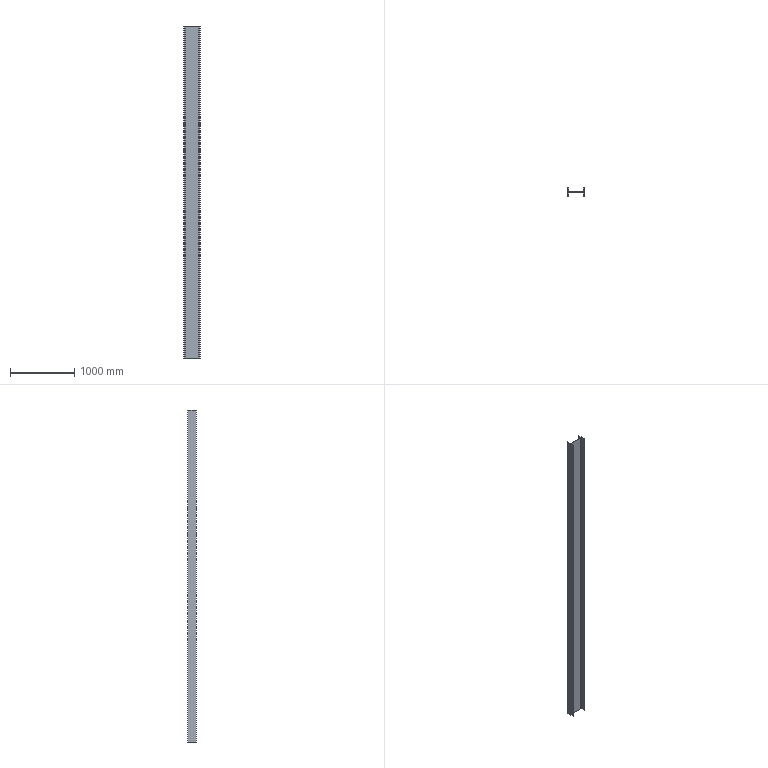Component | SolidWorks | H250X125-3800-1 | 1 solid | 18 faces | box 250 x 125 x 5180 mm | volume 19617027 mm3 | plane 14 | cylinder 4 | commonest cylinder face diameters 26 x4
build123d program:
from build123d import *

# Parameters (mm, degrees)
H_BEAM_HN250_125_1_DEPTH = 5180


with BuildPart() as part:
    # Sketch1 → H-Beam HN250_125_1 (new body)
    with BuildSketch(Plane.YZ):
        with BuildLine():
            Line((-62.5, -125), (-62.5, -116))
            Line((-62.5, -116), (-16, -116))
            ThreePointArc((-16, -116), (-6.808, -112.192), (-3, -103))
            Line((-3, -103), (-3, 103))
            ThreePointArc((-3, 103), (-6.808, 112.192), (-16, 116))
            Line((-16, 116), (-62.5, 116))
            Line((-62.5, 116), (-62.5, 125))
            Line((-62.5, 125), (62.5, 125))
            Line((62.5, 125), (62.5, 116))
            Line((62.5, 116), (16, 116))
            ThreePointArc((16, 116), (6.808, 112.192), (3, 103))
            Line((3, 103), (3, -103))
            ThreePointArc((3, -103), (6.808, -112.192), (16, -116))
            Line((16, -116), (62.5, -116))
            Line((62.5, -116), (62.5, -125))
            Line((62.5, -125), (-62.5, -125))
        make_face()
    extrude(amount=H_BEAM_HN250_125_1_DEPTH)


solid = part.part

# Placed as in the assembly
solid = solid.moved(Location((1944.926, 867.654, 5279), (0, 90, 0)))
STEP:
#1=COLOUR_RGB('',0.7922,0.8196,0.9333);
#2=FILL_AREA_STYLE_COLOUR('',#1);
#3=FILL_AREA_STYLE('',(#2));
#4=SURFACE_STYLE_FILL_AREA(#3);
#5=SURFACE_SIDE_STYLE('',(#4));
#6=SURFACE_STYLE_USAGE(.BOTH.,#5);
#7=PRESENTATION_STYLE_ASSIGNMENT((#6));
#8=CARTESIAN_POINT('',(71.651,31.699,207.835));
#9=VERTEX_POINT('',#8);
#10=CARTESIAN_POINT('',(71.651,36.62,207.835));
#11=VERTEX_POINT('',#10);
#12=CARTESIAN_POINT('',(71.651,36.62,207.835));
#13=DIRECTION('',(0.,1.,0.));
#14=VECTOR('',#13,39.37);
#15=LINE('',#12,#14);
#16=EDGE_CURVE('',#9,#11,#15,.T.);
#17=ORIENTED_EDGE('',*,*,#16,.T.);
#18=CARTESIAN_POINT('',(71.651,36.62,3.898));
#19=VERTEX_POINT('',#18);
#20=CARTESIAN_POINT('',(71.651,36.62,3.898));
#21=DIRECTION('',(0.,0.,1.));
#22=VECTOR('',#21,39.37);
#23=LINE('',#20,#22);
#24=EDGE_CURVE('',#19,#11,#23,.T.);
#25=ORIENTED_EDGE('',*,*,#24,.F.);
#26=CARTESIAN_POINT('',(71.651,31.699,3.898));
#27=VERTEX_POINT('',#26);
#28=CARTESIAN_POINT('',(71.651,36.62,3.898));
#29=DIRECTION('',(0.,1.,0.));
#30=VECTOR('',#29,39.37);
#31=LINE('',#28,#30);
#32=EDGE_CURVE('',#27,#19,#31,.T.);
#33=ORIENTED_EDGE('',*,*,#32,.F.);
#34=CARTESIAN_POINT('',(71.651,31.699,3.898));
#35=DIRECTION('',(0.,0.,1.));
#36=VECTOR('',#35,39.37);
#37=LINE('',#34,#36);
#38=EDGE_CURVE('',#27,#9,#37,.T.);
#39=ORIENTED_EDGE('',*,*,#38,.T.);
#40=EDGE_LOOP('',(#17,#25,#33,#39));
#41=FACE_OUTER_BOUND('',#40,.T.);
#42=CARTESIAN_POINT('',(71.651,36.62,3.898));
#43=DIRECTION('',(1.,0.,0.));
#44=DIRECTION('',(0.,0.,-1.));
#45=AXIS2_PLACEMENT_3D('',#42,#43,#44);
#46=PLANE('',#45);
#47=ADVANCED_FACE('',(#41),#46,.F.);
#48=CARTESIAN_POINT('',(72.005,36.62,207.835));
#49=VERTEX_POINT('',#48);
#50=CARTESIAN_POINT('',(72.005,36.62,207.835));
#51=DIRECTION('',(1.,0.,0.));
#52=VECTOR('',#51,39.37);
#53=LINE('',#50,#52);
#54=EDGE_CURVE('',#11,#49,#53,.T.);
#55=ORIENTED_EDGE('',*,*,#54,.T.);
#56=CARTESIAN_POINT('',(72.005,36.62,3.898));
#57=VERTEX_POINT('',#56);
#58=CARTESIAN_POINT('',(72.005,36.62,3.898));
#59=DIRECTION('',(0.,0.,1.));
#60=VECTOR('',#59,39.37);
#61=LINE('',#58,#60);
#62=EDGE_CURVE('',#57,#49,#61,.T.);
#63=ORIENTED_EDGE('',*,*,#62,.F.);
#64=CARTESIAN_POINT('',(72.005,36.62,3.898));
#65=DIRECTION('',(1.,0.,0.));
#66=VECTOR('',#65,39.37);
#67=LINE('',#64,#66);
#68=EDGE_CURVE('',#19,#57,#67,.T.);
#69=ORIENTED_EDGE('',*,*,#68,.F.);
#70=ORIENTED_EDGE('',*,*,#24,.T.);
#71=EDGE_LOOP('',(#55,#63,#69,#70));
#72=FACE_OUTER_BOUND('',#71,.T.);
#73=CARTESIAN_POINT('',(72.005,36.62,3.898));
#74=DIRECTION('',(0.,-1.,0.));
#75=DIRECTION('',(-1.,0.,0.));
#76=AXIS2_PLACEMENT_3D('',#73,#74,#75);
#77=PLANE('',#76);
#78=ADVANCED_FACE('',(#72),#77,.F.);
#79=CARTESIAN_POINT('',(72.005,34.79,207.835));
#80=VERTEX_POINT('',#79);
#81=CARTESIAN_POINT('',(72.005,36.62,207.835));
#82=DIRECTION('',(0.,-1.,0.));
#83=VECTOR('',#82,39.37);
#84=LINE('',#81,#83);
#85=EDGE_CURVE('',#49,#80,#84,.T.);
#86=ORIENTED_EDGE('',*,*,#85,.T.);
#87=CARTESIAN_POINT('',(72.005,34.79,3.898));
#88=VERTEX_POINT('',#87);
#89=CARTESIAN_POINT('',(72.005,34.79,3.898));
#90=DIRECTION('',(0.,0.,1.));
#91=VECTOR('',#90,39.37);
#92=LINE('',#89,#91);
#93=EDGE_CURVE('',#88,#80,#92,.T.);
#94=ORIENTED_EDGE('',*,*,#93,.F.);
#95=CARTESIAN_POINT('',(72.005,36.62,3.898));
#96=DIRECTION('',(0.,-1.,0.));
#97=VECTOR('',#96,39.37);
#98=LINE('',#95,#97);
#99=EDGE_CURVE('',#57,#88,#98,.T.);
#100=ORIENTED_EDGE('',*,*,#99,.F.);
#101=ORIENTED_EDGE('',*,*,#62,.T.);
#102=EDGE_LOOP('',(#86,#94,#100,#101));
#103=FACE_OUTER_BOUND('',#102,.T.);
#104=CARTESIAN_POINT('',(72.005,36.62,3.898));
#105=DIRECTION('',(-1.,-0.,0.));
#106=DIRECTION('',(-0.,1.,0.));
#107=AXIS2_PLACEMENT_3D('',#104,#105,#106);
#108=PLANE('',#107);
#109=ADVANCED_FACE('',(#103),#108,.F.);
#110=CARTESIAN_POINT('',(72.517,34.278,207.835));
#111=VERTEX_POINT('',#110);
#112=CARTESIAN_POINT('',(72.517,34.79,207.835));
#113=DIRECTION('',(0.,0.,1.));
#114=DIRECTION('',(1.,0.,0.));
#115=AXIS2_PLACEMENT_3D('',#112,#113,#114);
#116=CIRCLE('',#115,0.5118);
#117=EDGE_CURVE('',#80,#111,#116,.T.);
#118=ORIENTED_EDGE('',*,*,#117,.T.);
#119=CARTESIAN_POINT('',(72.517,34.278,3.898));
#120=VERTEX_POINT('',#119);
#121=CARTESIAN_POINT('',(72.517,34.278,3.898));
#122=DIRECTION('',(0.,0.,1.));
#123=VECTOR('',#122,39.37);
#124=LINE('',#121,#123);
#125=EDGE_CURVE('',#120,#111,#124,.T.);
#126=ORIENTED_EDGE('',*,*,#125,.F.);
#127=CARTESIAN_POINT('',(72.517,34.79,3.898));
#128=DIRECTION('',(0.,0.,1.));
#129=DIRECTION('',(1.,0.,0.));
#130=AXIS2_PLACEMENT_3D('',#127,#128,#129);
#131=CIRCLE('',#130,0.5118);
#132=EDGE_CURVE('',#88,#120,#131,.T.);
#133=ORIENTED_EDGE('',*,*,#132,.F.);
#134=ORIENTED_EDGE('',*,*,#93,.T.);
#135=EDGE_LOOP('',(#118,#126,#133,#134));
#136=FACE_OUTER_BOUND('',#135,.T.);
#137=CARTESIAN_POINT('',(72.517,34.79,3.898));
#138=DIRECTION('',(0.,0.,1.));
#139=DIRECTION('',(1.,0.,0.));
#140=AXIS2_PLACEMENT_3D('',#137,#138,#139);
#141=CYLINDRICAL_SURFACE('',#140,0.5118);
#142=ADVANCED_FACE('',(#136),#141,.F.);
#143=CARTESIAN_POINT('',(80.627,34.278,207.835));
#144=VERTEX_POINT('',#143);
#145=CARTESIAN_POINT('',(80.627,34.278,207.835));
#146=DIRECTION('',(1.,-0.,0.));
#147=VECTOR('',#146,39.37);
#148=LINE('',#145,#147);
#149=EDGE_CURVE('',#111,#144,#148,.T.);
#150=ORIENTED_EDGE('',*,*,#149,.T.);
#151=CARTESIAN_POINT('',(80.627,34.278,3.898));
#152=VERTEX_POINT('',#151);
#153=CARTESIAN_POINT('',(80.627,34.278,3.898));
#154=DIRECTION('',(0.,0.,1.));
#155=VECTOR('',#154,39.37);
#156=LINE('',#153,#155);
#157=EDGE_CURVE('',#152,#144,#156,.T.);
#158=ORIENTED_EDGE('',*,*,#157,.F.);
#159=CARTESIAN_POINT('',(80.627,34.278,3.898));
#160=DIRECTION('',(1.,-0.,0.));
#161=VECTOR('',#160,39.37);
#162=LINE('',#159,#161);
#163=EDGE_CURVE('',#120,#152,#162,.T.);
#164=ORIENTED_EDGE('',*,*,#163,.F.);
#165=ORIENTED_EDGE('',*,*,#125,.T.);
#166=EDGE_LOOP('',(#150,#158,#164,#165));
#167=FACE_OUTER_BOUND('',#166,.T.);
#168=CARTESIAN_POINT('',(80.627,34.278,3.898));
#169=DIRECTION('',(-0.,-1.,0.));
#170=DIRECTION('',(-1.,0.,0.));
#171=AXIS2_PLACEMENT_3D('',#168,#169,#170);
#172=PLANE('',#171);
#173=ADVANCED_FACE('',(#167),#172,.F.);
#174=CARTESIAN_POINT('',(81.139,34.79,207.835));
#175=VERTEX_POINT('',#174);
#176=CARTESIAN_POINT('',(80.627,34.79,207.835));
#177=DIRECTION('',(0.,0.,1.));
#178=DIRECTION('',(1.,0.,0.));
#179=AXIS2_PLACEMENT_3D('',#176,#177,#178);
#180=CIRCLE('',#179,0.5118);
#181=EDGE_CURVE('',#144,#175,#180,.T.);
#182=ORIENTED_EDGE('',*,*,#181,.T.);
#183=CARTESIAN_POINT('',(81.139,34.79,3.898));
#184=VERTEX_POINT('',#183);
#185=CARTESIAN_POINT('',(81.139,34.79,3.898));
#186=DIRECTION('',(0.,0.,1.));
#187=VECTOR('',#186,39.37);
#188=LINE('',#185,#187);
#189=EDGE_CURVE('',#184,#175,#188,.T.);
#190=ORIENTED_EDGE('',*,*,#189,.F.);
#191=CARTESIAN_POINT('',(80.627,34.79,3.898));
#192=DIRECTION('',(0.,0.,1.));
#193=DIRECTION('',(1.,0.,0.));
#194=AXIS2_PLACEMENT_3D('',#191,#192,#193);
#195=CIRCLE('',#194,0.5118);
#196=EDGE_CURVE('',#152,#184,#195,.T.);
#197=ORIENTED_EDGE('',*,*,#196,.F.);
#198=ORIENTED_EDGE('',*,*,#157,.T.);
#199=EDGE_LOOP('',(#182,#190,#197,#198));
#200=FACE_OUTER_BOUND('',#199,.T.);
#201=CARTESIAN_POINT('',(80.627,34.79,3.898));
#202=DIRECTION('',(0.,0.,1.));
#203=DIRECTION('',(1.,0.,0.));
#204=AXIS2_PLACEMENT_3D('',#201,#202,#203);
#205=CYLINDRICAL_SURFACE('',#204,0.5118);
#206=ADVANCED_FACE('',(#200),#205,.F.);
#207=CARTESIAN_POINT('',(81.139,36.62,207.835));
#208=VERTEX_POINT('',#207);
#209=CARTESIAN_POINT('',(81.139,34.79,207.835));
#210=DIRECTION('',(0.,1.,0.));
#211=VECTOR('',#210,39.37);
#212=LINE('',#209,#211);
#213=EDGE_CURVE('',#175,#208,#212,.T.);
#214=ORIENTED_EDGE('',*,*,#213,.T.);
#215=CARTESIAN_POINT('',(81.139,36.62,3.898));
#216=VERTEX_POINT('',#215);
#217=CARTESIAN_POINT('',(81.139,36.62,3.898));
#218=DIRECTION('',(0.,0.,1.));
#219=VECTOR('',#218,39.37);
#220=LINE('',#217,#219);
#221=EDGE_CURVE('',#216,#208,#220,.T.);
#222=ORIENTED_EDGE('',*,*,#221,.F.);
#223=CARTESIAN_POINT('',(81.139,34.79,3.898));
#224=DIRECTION('',(0.,1.,0.));
#225=VECTOR('',#224,39.37);
#226=LINE('',#223,#225);
#227=EDGE_CURVE('',#184,#216,#226,.T.);
#228=ORIENTED_EDGE('',*,*,#227,.F.);
#229=ORIENTED_EDGE('',*,*,#189,.T.);
#230=EDGE_LOOP('',(#214,#222,#228,#229));
#231=FACE_OUTER_BOUND('',#230,.T.);
#232=CARTESIAN_POINT('',(81.139,34.79,3.898));
#233=DIRECTION('',(1.,0.,0.));
#234=DIRECTION('',(0.,0.,-1.));
#235=AXIS2_PLACEMENT_3D('',#232,#233,#234);
#236=PLANE('',#235);
#237=ADVANCED_FACE('',(#231),#236,.F.);
#238=CARTESIAN_POINT('',(81.493,36.62,207.835));
#239=VERTEX_POINT('',#238);
#240=CARTESIAN_POINT('',(81.493,36.62,207.835));
#241=DIRECTION('',(1.,0.,0.));
#242=VECTOR('',#241,39.37);
#243=LINE('',#240,#242);
#244=EDGE_CURVE('',#208,#239,#243,.T.);
#245=ORIENTED_EDGE('',*,*,#244,.T.);
#246=CARTESIAN_POINT('',(81.493,36.62,3.898));
#247=VERTEX_POINT('',#246);
#248=CARTESIAN_POINT('',(81.493,36.62,3.898));
#249=DIRECTION('',(0.,0.,1.));
#250=VECTOR('',#249,39.37);
#251=LINE('',#248,#250);
#252=EDGE_CURVE('',#247,#239,#251,.T.);
#253=ORIENTED_EDGE('',*,*,#252,.F.);
#254=CARTESIAN_POINT('',(81.493,36.62,3.898));
#255=DIRECTION('',(1.,0.,0.));
#256=VECTOR('',#255,39.37);
#257=LINE('',#254,#256);
#258=EDGE_CURVE('',#216,#247,#257,.T.);
#259=ORIENTED_EDGE('',*,*,#258,.F.);
#260=ORIENTED_EDGE('',*,*,#221,.T.);
#261=EDGE_LOOP('',(#245,#253,#259,#260));
#262=FACE_OUTER_BOUND('',#261,.T.);
#263=CARTESIAN_POINT('',(81.493,36.62,3.898));
#264=DIRECTION('',(0.,-1.,0.));
#265=DIRECTION('',(-1.,0.,0.));
#266=AXIS2_PLACEMENT_3D('',#263,#264,#265);
#267=PLANE('',#266);
#268=ADVANCED_FACE('',(#262),#267,.F.);
#269=CARTESIAN_POINT('',(81.493,31.699,207.835));
#270=VERTEX_POINT('',#269);
#271=CARTESIAN_POINT('',(81.493,31.699,207.835));
#272=DIRECTION('',(0.,-1.,0.));
#273=VECTOR('',#272,39.37);
#274=LINE('',#271,#273);
#275=EDGE_CURVE('',#239,#270,#274,.T.);
#276=ORIENTED_EDGE('',*,*,#275,.T.);
#277=CARTESIAN_POINT('',(81.493,31.699,3.898));
#278=VERTEX_POINT('',#277);
#279=CARTESIAN_POINT('',(81.493,31.699,3.898));
#280=DIRECTION('',(0.,0.,1.));
#281=VECTOR('',#280,39.37);
#282=LINE('',#279,#281);
#283=EDGE_CURVE('',#278,#270,#282,.T.);
#284=ORIENTED_EDGE('',*,*,#283,.F.);
#285=CARTESIAN_POINT('',(81.493,31.699,3.898));
#286=DIRECTION('',(0.,-1.,0.));
#287=VECTOR('',#286,39.37);
#288=LINE('',#285,#287);
#289=EDGE_CURVE('',#247,#278,#288,.T.);
#290=ORIENTED_EDGE('',*,*,#289,.F.);
#291=ORIENTED_EDGE('',*,*,#252,.T.);
#292=EDGE_LOOP('',(#276,#284,#290,#291));
#293=FACE_OUTER_BOUND('',#292,.T.);
#294=CARTESIAN_POINT('',(81.493,31.699,3.898));
#295=DIRECTION('',(-1.,0.,0.));
#296=DIRECTION('',(0.,0.,1.));
#297=AXIS2_PLACEMENT_3D('',#294,#295,#296);
#298=PLANE('',#297);
#299=ADVANCED_FACE('',(#293),#298,.F.);
#300=CARTESIAN_POINT('',(81.139,31.699,207.835));
#301=VERTEX_POINT('',#300);
#302=CARTESIAN_POINT('',(81.139,31.699,207.835));
#303=DIRECTION('',(-1.,0.,0.));
#304=VECTOR('',#303,39.37);
#305=LINE('',#302,#304);
#306=EDGE_CURVE('',#270,#301,#305,.T.);
#307=ORIENTED_EDGE('',*,*,#306,.T.);
#308=CARTESIAN_POINT('',(81.139,31.699,3.898));
#309=VERTEX_POINT('',#308);
#310=CARTESIAN_POINT('',(81.139,31.699,3.898));
#311=DIRECTION('',(0.,0.,1.));
#312=VECTOR('',#311,39.37);
#313=LINE('',#310,#312);
#314=EDGE_CURVE('',#309,#301,#313,.T.);
#315=ORIENTED_EDGE('',*,*,#314,.F.);
#316=CARTESIAN_POINT('',(81.139,31.699,3.898));
#317=DIRECTION('',(-1.,0.,0.));
#318=VECTOR('',#317,39.37);
#319=LINE('',#316,#318);
#320=EDGE_CURVE('',#278,#309,#319,.T.);
#321=ORIENTED_EDGE('',*,*,#320,.F.);
#322=ORIENTED_EDGE('',*,*,#283,.T.);
#323=EDGE_LOOP('',(#307,#315,#321,#322));
#324=FACE_OUTER_BOUND('',#323,.T.);
#325=CARTESIAN_POINT('',(81.139,31.699,3.898));
#326=DIRECTION('',(0.,1.,0.));
#327=DIRECTION('',(1.,0.,0.));
#328=AXIS2_PLACEMENT_3D('',#325,#326,#327);
#329=PLANE('',#328);
#330=ADVANCED_FACE('',(#324),#329,.F.);
#331=CARTESIAN_POINT('',(81.139,33.53,207.835));
#332=VERTEX_POINT('',#331);
#333=CARTESIAN_POINT('',(81.139,31.699,207.835));
#334=DIRECTION('',(0.,1.,0.));
#335=VECTOR('',#334,39.37);
#336=LINE('',#333,#335);
#337=EDGE_CURVE('',#301,#332,#336,.T.);
#338=ORIENTED_EDGE('',*,*,#337,.T.);
#339=CARTESIAN_POINT('',(81.139,33.53,3.898));
#340=VERTEX_POINT('',#339);
#341=CARTESIAN_POINT('',(81.139,33.53,3.898));
#342=DIRECTION('',(0.,0.,1.));
#343=VECTOR('',#342,39.37);
#344=LINE('',#341,#343);
#345=EDGE_CURVE('',#340,#332,#344,.T.);
#346=ORIENTED_EDGE('',*,*,#345,.F.);
#347=CARTESIAN_POINT('',(81.139,31.699,3.898));
#348=DIRECTION('',(0.,1.,0.));
#349=VECTOR('',#348,39.37);
#350=LINE('',#347,#349);
#351=EDGE_CURVE('',#309,#340,#350,.T.);
#352=ORIENTED_EDGE('',*,*,#351,.F.);
#353=ORIENTED_EDGE('',*,*,#314,.T.);
#354=EDGE_LOOP('',(#338,#346,#352,#353));
#355=FACE_OUTER_BOUND('',#354,.T.);
#356=CARTESIAN_POINT('',(81.139,31.699,3.898));
#357=DIRECTION('',(1.,0.,0.));
#358=DIRECTION('',(0.,0.,-1.));
#359=AXIS2_PLACEMENT_3D('',#356,#357,#358);
#360=PLANE('',#359);
#361=ADVANCED_FACE('',(#355),#360,.F.);
#362=CARTESIAN_POINT('',(80.627,34.041,207.835));
#363=VERTEX_POINT('',#362);
#364=CARTESIAN_POINT('',(80.627,33.53,207.835));
#365=DIRECTION('',(0.,0.,1.));
#366=DIRECTION('',(-1.,0.,0.));
#367=AXIS2_PLACEMENT_3D('',#364,#365,#366);
#368=CIRCLE('',#367,0.5118);
#369=EDGE_CURVE('',#332,#363,#368,.T.);
#370=ORIENTED_EDGE('',*,*,#369,.T.);
#371=CARTESIAN_POINT('',(80.627,34.041,3.898));
#372=VERTEX_POINT('',#371);
#373=CARTESIAN_POINT('',(80.627,34.041,3.898));
#374=DIRECTION('',(0.,0.,1.));
#375=VECTOR('',#374,39.37);
#376=LINE('',#373,#375);
#377=EDGE_CURVE('',#372,#363,#376,.T.);
#378=ORIENTED_EDGE('',*,*,#377,.F.);
#379=CARTESIAN_POINT('',(80.627,33.53,3.898));
#380=DIRECTION('',(0.,0.,1.));
#381=DIRECTION('',(-1.,0.,0.));
#382=AXIS2_PLACEMENT_3D('',#379,#380,#381);
#383=CIRCLE('',#382,0.5118);
#384=EDGE_CURVE('',#340,#372,#383,.T.);
#385=ORIENTED_EDGE('',*,*,#384,.F.);
#386=ORIENTED_EDGE('',*,*,#345,.T.);
#387=EDGE_LOOP('',(#370,#378,#385,#386));
#388=FACE_OUTER_BOUND('',#387,.T.);
#389=CARTESIAN_POINT('',(80.627,33.53,3.898));
#390=DIRECTION('',(0.,0.,1.));
#391=DIRECTION('',(1.,0.,0.));
#392=AXIS2_PLACEMENT_3D('',#389,#390,#391);
#393=CYLINDRICAL_SURFACE('',#392,0.5118);
#394=ADVANCED_FACE('',(#388),#393,.F.);
#395=CARTESIAN_POINT('',(72.517,34.041,207.835));
#396=VERTEX_POINT('',#395);
#397=CARTESIAN_POINT('',(72.517,34.041,207.835));
#398=DIRECTION('',(-1.,0.,0.));
#399=VECTOR('',#398,39.37);
#400=LINE('',#397,#399);
#401=EDGE_CURVE('',#363,#396,#400,.T.);
#402=ORIENTED_EDGE('',*,*,#401,.T.);
#403=CARTESIAN_POINT('',(72.517,34.041,3.898));
#404=VERTEX_POINT('',#403);
#405=CARTESIAN_POINT('',(72.517,34.041,3.898));
#406=DIRECTION('',(0.,0.,1.));
#407=VECTOR('',#406,39.37);
#408=LINE('',#405,#407);
#409=EDGE_CURVE('',#404,#396,#408,.T.);
#410=ORIENTED_EDGE('',*,*,#409,.F.);
#411=CARTESIAN_POINT('',(72.517,34.041,3.898));
#412=DIRECTION('',(-1.,0.,0.));
#413=VECTOR('',#412,39.37);
#414=LINE('',#411,#413);
#415=EDGE_CURVE('',#372,#404,#414,.T.);
#416=ORIENTED_EDGE('',*,*,#415,.F.);
#417=ORIENTED_EDGE('',*,*,#377,.T.);
#418=EDGE_LOOP('',(#402,#410,#416,#417));
#419=FACE_OUTER_BOUND('',#418,.T.);
#420=CARTESIAN_POINT('',(72.517,34.041,3.898));
#421=DIRECTION('',(0.,1.,0.));
#422=DIRECTION('',(1.,-0.,0.));
#423=AXIS2_PLACEMENT_3D('',#420,#421,#422);
#424=PLANE('',#423);
#425=ADVANCED_FACE('',(#419),#424,.F.);
#426=CARTESIAN_POINT('',(72.005,33.53,207.835));
#427=VERTEX_POINT('',#426);
#428=CARTESIAN_POINT('',(72.517,33.53,207.835));
#429=DIRECTION('',(0.,0.,1.));
#430=DIRECTION('',(-1.,0.,0.));
#431=AXIS2_PLACEMENT_3D('',#428,#429,#430);
#432=CIRCLE('',#431,0.5118);
#433=EDGE_CURVE('',#396,#427,#432,.T.);
#434=ORIENTED_EDGE('',*,*,#433,.T.);
#435=CARTESIAN_POINT('',(72.005,33.53,3.898));
#436=VERTEX_POINT('',#435);
#437=CARTESIAN_POINT('',(72.005,33.53,3.898));
#438=DIRECTION('',(0.,0.,1.));
#439=VECTOR('',#438,39.37);
#440=LINE('',#437,#439);
#441=EDGE_CURVE('',#436,#427,#440,.T.);
#442=ORIENTED_EDGE('',*,*,#441,.F.);
#443=CARTESIAN_POINT('',(72.517,33.53,3.898));
#444=DIRECTION('',(0.,0.,1.));
#445=DIRECTION('',(-1.,0.,0.));
#446=AXIS2_PLACEMENT_3D('',#443,#444,#445);
#447=CIRCLE('',#446,0.5118);
#448=EDGE_CURVE('',#404,#436,#447,.T.);
#449=ORIENTED_EDGE('',*,*,#448,.F.);
#450=ORIENTED_EDGE('',*,*,#409,.T.);
#451=EDGE_LOOP('',(#434,#442,#449,#450));
#452=FACE_OUTER_BOUND('',#451,.T.);
#453=CARTESIAN_POINT('',(72.517,33.53,3.898));
#454=DIRECTION('',(0.,0.,1.));
#455=DIRECTION('',(1.,0.,0.));
#456=AXIS2_PLACEMENT_3D('',#453,#454,#455);
#457=CYLINDRICAL_SURFACE('',#456,0.5118);
#458=ADVANCED_FACE('',(#452),#457,.F.);
#459=CARTESIAN_POINT('',(72.005,31.699,207.835));
#460=VERTEX_POINT('',#459);
#461=CARTESIAN_POINT('',(72.005,33.53,207.835));
#462=DIRECTION('',(-0.,-1.,0.));
#463=VECTOR('',#462,39.37);
#464=LINE('',#461,#463);
#465=EDGE_CURVE('',#427,#460,#464,.T.);
#466=ORIENTED_EDGE('',*,*,#465,.T.);
#467=CARTESIAN_POINT('',(72.005,31.699,3.898));
#468=VERTEX_POINT('',#467);
#469=CARTESIAN_POINT('',(72.005,31.699,3.898));
#470=DIRECTION('',(0.,0.,1.));
#471=VECTOR('',#470,39.37);
#472=LINE('',#469,#471);
#473=EDGE_CURVE('',#468,#460,#472,.T.);
#474=ORIENTED_EDGE('',*,*,#473,.F.);
#475=CARTESIAN_POINT('',(72.005,33.53,3.898));
#476=DIRECTION('',(-0.,-1.,0.));
#477=VECTOR('',#476,39.37);
#478=LINE('',#475,#477);
#479=EDGE_CURVE('',#436,#468,#478,.T.);
#480=ORIENTED_EDGE('',*,*,#479,.F.);
#481=ORIENTED_EDGE('',*,*,#441,.T.);
#482=EDGE_LOOP('',(#466,#474,#480,#481));
#483=FACE_OUTER_BOUND('',#482,.T.);
#484=CARTESIAN_POINT('',(72.005,33.53,3.898));
#485=DIRECTION('',(-1.,0.,0.));
#486=DIRECTION('',(0.,1.,0.));
#487=AXIS2_PLACEMENT_3D('',#484,#485,#486);
#488=PLANE('',#487);
#489=ADVANCED_FACE('',(#483),#488,.F.);
#490=CARTESIAN_POINT('',(71.651,31.699,207.835));
#491=DIRECTION('',(-1.,0.,0.));
#492=VECTOR('',#491,39.37);
#493=LINE('',#490,#492);
#494=EDGE_CURVE('',#460,#9,#493,.T.);
#495=ORIENTED_EDGE('',*,*,#494,.T.);
#496=ORIENTED_EDGE('',*,*,#38,.F.);
#497=CARTESIAN_POINT('',(71.651,31.699,3.898));
#498=DIRECTION('',(-1.,0.,0.));
#499=VECTOR('',#498,39.37);
#500=LINE('',#497,#499);
#501=EDGE_CURVE('',#468,#27,#500,.T.);
#502=ORIENTED_EDGE('',*,*,#501,.F.);
#503=ORIENTED_EDGE('',*,*,#473,.T.);
#504=EDGE_LOOP('',(#495,#496,#502,#503));
#505=FACE_OUTER_BOUND('',#504,.T.);
#506=CARTESIAN_POINT('',(71.651,31.699,3.898));
#507=DIRECTION('',(0.,1.,0.));
#508=DIRECTION('',(1.,0.,0.));
#509=AXIS2_PLACEMENT_3D('',#506,#507,#508);
#510=PLANE('',#509);
#511=ADVANCED_FACE('',(#505),#510,.F.);
#512=ORIENTED_EDGE('',*,*,#32,.T.);
#513=ORIENTED_EDGE('',*,*,#68,.T.);
#514=ORIENTED_EDGE('',*,*,#99,.T.);
#515=ORIENTED_EDGE('',*,*,#132,.T.);
#516=ORIENTED_EDGE('',*,*,#163,.T.);
#517=ORIENTED_EDGE('',*,*,#196,.T.);
#518=ORIENTED_EDGE('',*,*,#227,.T.);
#519=ORIENTED_EDGE('',*,*,#258,.T.);
#520=ORIENTED_EDGE('',*,*,#289,.T.);
#521=ORIENTED_EDGE('',*,*,#320,.T.);
#522=ORIENTED_EDGE('',*,*,#351,.T.);
#523=ORIENTED_EDGE('',*,*,#384,.T.);
#524=ORIENTED_EDGE('',*,*,#415,.T.);
#525=ORIENTED_EDGE('',*,*,#448,.T.);
#526=ORIENTED_EDGE('',*,*,#479,.T.);
#527=ORIENTED_EDGE('',*,*,#501,.T.);
#528=EDGE_LOOP('',(#512,#513,#514,#515,#516,#517,#518,#519,#520,#521,#522,#523,#524,#525,#526,#527));
#529=FACE_OUTER_BOUND('',#528,.T.);
#530=CARTESIAN_POINT('',(72.517,33.53,3.898));
#531=DIRECTION('',(0.,0.,-1.));
#532=DIRECTION('',(-1.,0.,0.));
#533=AXIS2_PLACEMENT_3D('',#530,#531,#532);
#534=PLANE('',#533);
#535=ADVANCED_FACE('',(#529),#534,.T.);
#536=ORIENTED_EDGE('',*,*,#16,.F.);
#537=ORIENTED_EDGE('',*,*,#494,.F.);
#538=ORIENTED_EDGE('',*,*,#465,.F.);
#539=ORIENTED_EDGE('',*,*,#433,.F.);
#540=ORIENTED_EDGE('',*,*,#401,.F.);
#541=ORIENTED_EDGE('',*,*,#369,.F.);
#542=ORIENTED_EDGE('',*,*,#337,.F.);
#543=ORIENTED_EDGE('',*,*,#306,.F.);
#544=ORIENTED_EDGE('',*,*,#275,.F.);
#545=ORIENTED_EDGE('',*,*,#244,.F.);
#546=ORIENTED_EDGE('',*,*,#213,.F.);
#547=ORIENTED_EDGE('',*,*,#181,.F.);
#548=ORIENTED_EDGE('',*,*,#149,.F.);
#549=ORIENTED_EDGE('',*,*,#117,.F.);
#550=ORIENTED_EDGE('',*,*,#85,.F.);
#551=ORIENTED_EDGE('',*,*,#54,.F.);
#552=EDGE_LOOP('',(#536,#537,#538,#539,#540,#541,#542,#543,#544,#545,#546,#547,#548,#549,#550,#551));
#553=FACE_OUTER_BOUND('',#552,.T.);
#554=CARTESIAN_POINT('',(72.517,33.53,207.835));
#555=DIRECTION('',(0.,0.,-1.));
#556=DIRECTION('',(-1.,0.,0.));
#557=AXIS2_PLACEMENT_3D('',#554,#555,#556);
#558=PLANE('',#557);
#559=ADVANCED_FACE('',(#553),#558,.F.);
#560=CLOSED_SHELL('',(#47,#78,#109,#142,#173,#206,#237,#268,#299,#330,#361,#394,#425,#458,#489,#511,#535,#559));
#561=MANIFOLD_SOLID_BREP('',#560);
#562=STYLED_ITEM('',(#7),#561);
#563=(LENGTH_UNIT()NAMED_UNIT(*)SI_UNIT($,.METRE.));
#564=LENGTH_MEASURE_WITH_UNIT(LENGTH_MEASURE(0.0254),#563);
#565=DIMENSIONAL_EXPONENTS(1.,0.,0.,0.,0.,0.,0.);
#566=(CONVERSION_BASED_UNIT('',#564)LENGTH_UNIT()NAMED_UNIT(#565));
#567=UNCERTAINTY_MEASURE_WITH_UNIT(LENGTH_MEASURE(0.00001),#566,'','');
#568=(NAMED_UNIT(*)PLANE_ANGLE_UNIT()SI_UNIT($,.RADIAN.));
#569=(NAMED_UNIT(*)SI_UNIT($,.STERADIAN.)SOLID_ANGLE_UNIT());
#570=(GEOMETRIC_REPRESENTATION_CONTEXT(3)GLOBAL_UNCERTAINTY_ASSIGNED_CONTEXT((#567))GLOBAL_UNIT_ASSIGNED_CONTEXT((#566,#568,#569))REPRESENTATION_CONTEXT('',''));
#571=MECHANICAL_DESIGN_GEOMETRIC_PRESENTATION_REPRESENTATION('',(#562),#570);
#572=PRESENTATION_LAYER_ASSIGNMENT('','',(#562));
#573=CARTESIAN_POINT('',(0.,0.,0.));
#574=DIRECTION('',(0.,0.,1.));
#575=DIRECTION('',(1.,0.,0.));
#576=AXIS2_PLACEMENT_3D('',#573,#574,#575);
#577=(LENGTH_UNIT()NAMED_UNIT(*)SI_UNIT($,.METRE.));
#578=LENGTH_MEASURE_WITH_UNIT(LENGTH_MEASURE(0.0254),#577);
#579=DIMENSIONAL_EXPONENTS(1.,0.,0.,0.,0.,0.,0.);
#580=(CONVERSION_BASED_UNIT('',#578)LENGTH_UNIT()NAMED_UNIT(#579));
#581=UNCERTAINTY_MEASURE_WITH_UNIT(LENGTH_MEASURE(0.00001),#580,'','');
#582=(NAMED_UNIT(*)PLANE_ANGLE_UNIT()SI_UNIT($,.RADIAN.));
#583=(NAMED_UNIT(*)SI_UNIT($,.STERADIAN.)SOLID_ANGLE_UNIT());
#584=(GEOMETRIC_REPRESENTATION_CONTEXT(3)GLOBAL_UNCERTAINTY_ASSIGNED_CONTEXT((#581))GLOBAL_UNIT_ASSIGNED_CONTEXT((#580,#582,#583))REPRESENTATION_CONTEXT('',''));
#585=ADVANCED_BREP_SHAPE_REPRESENTATION('',(#561,#576),#584);